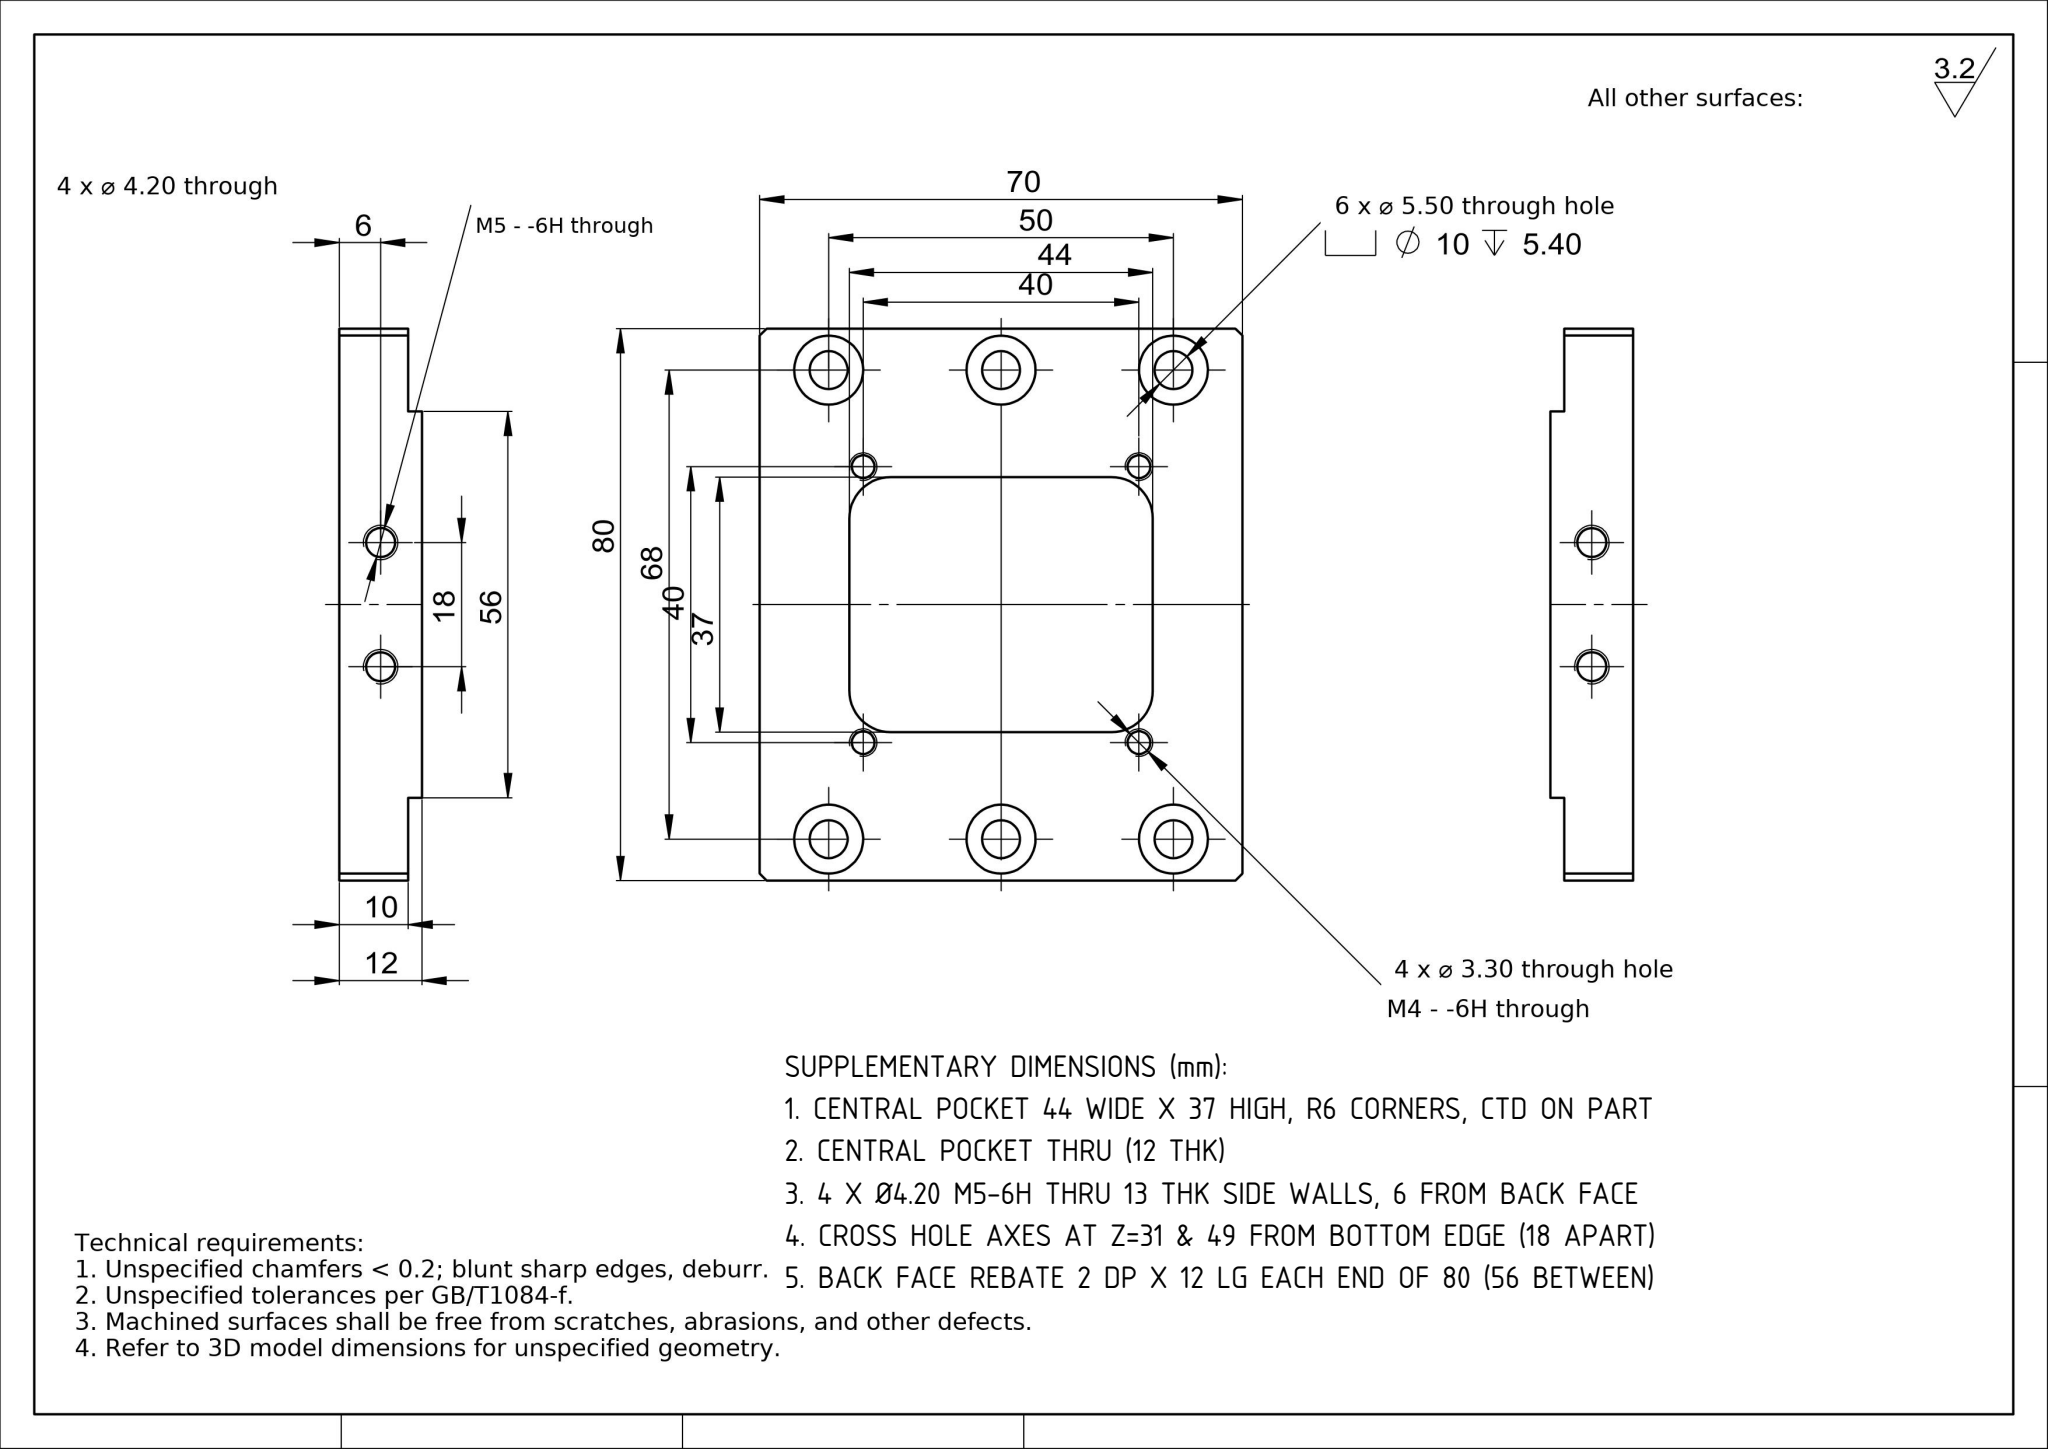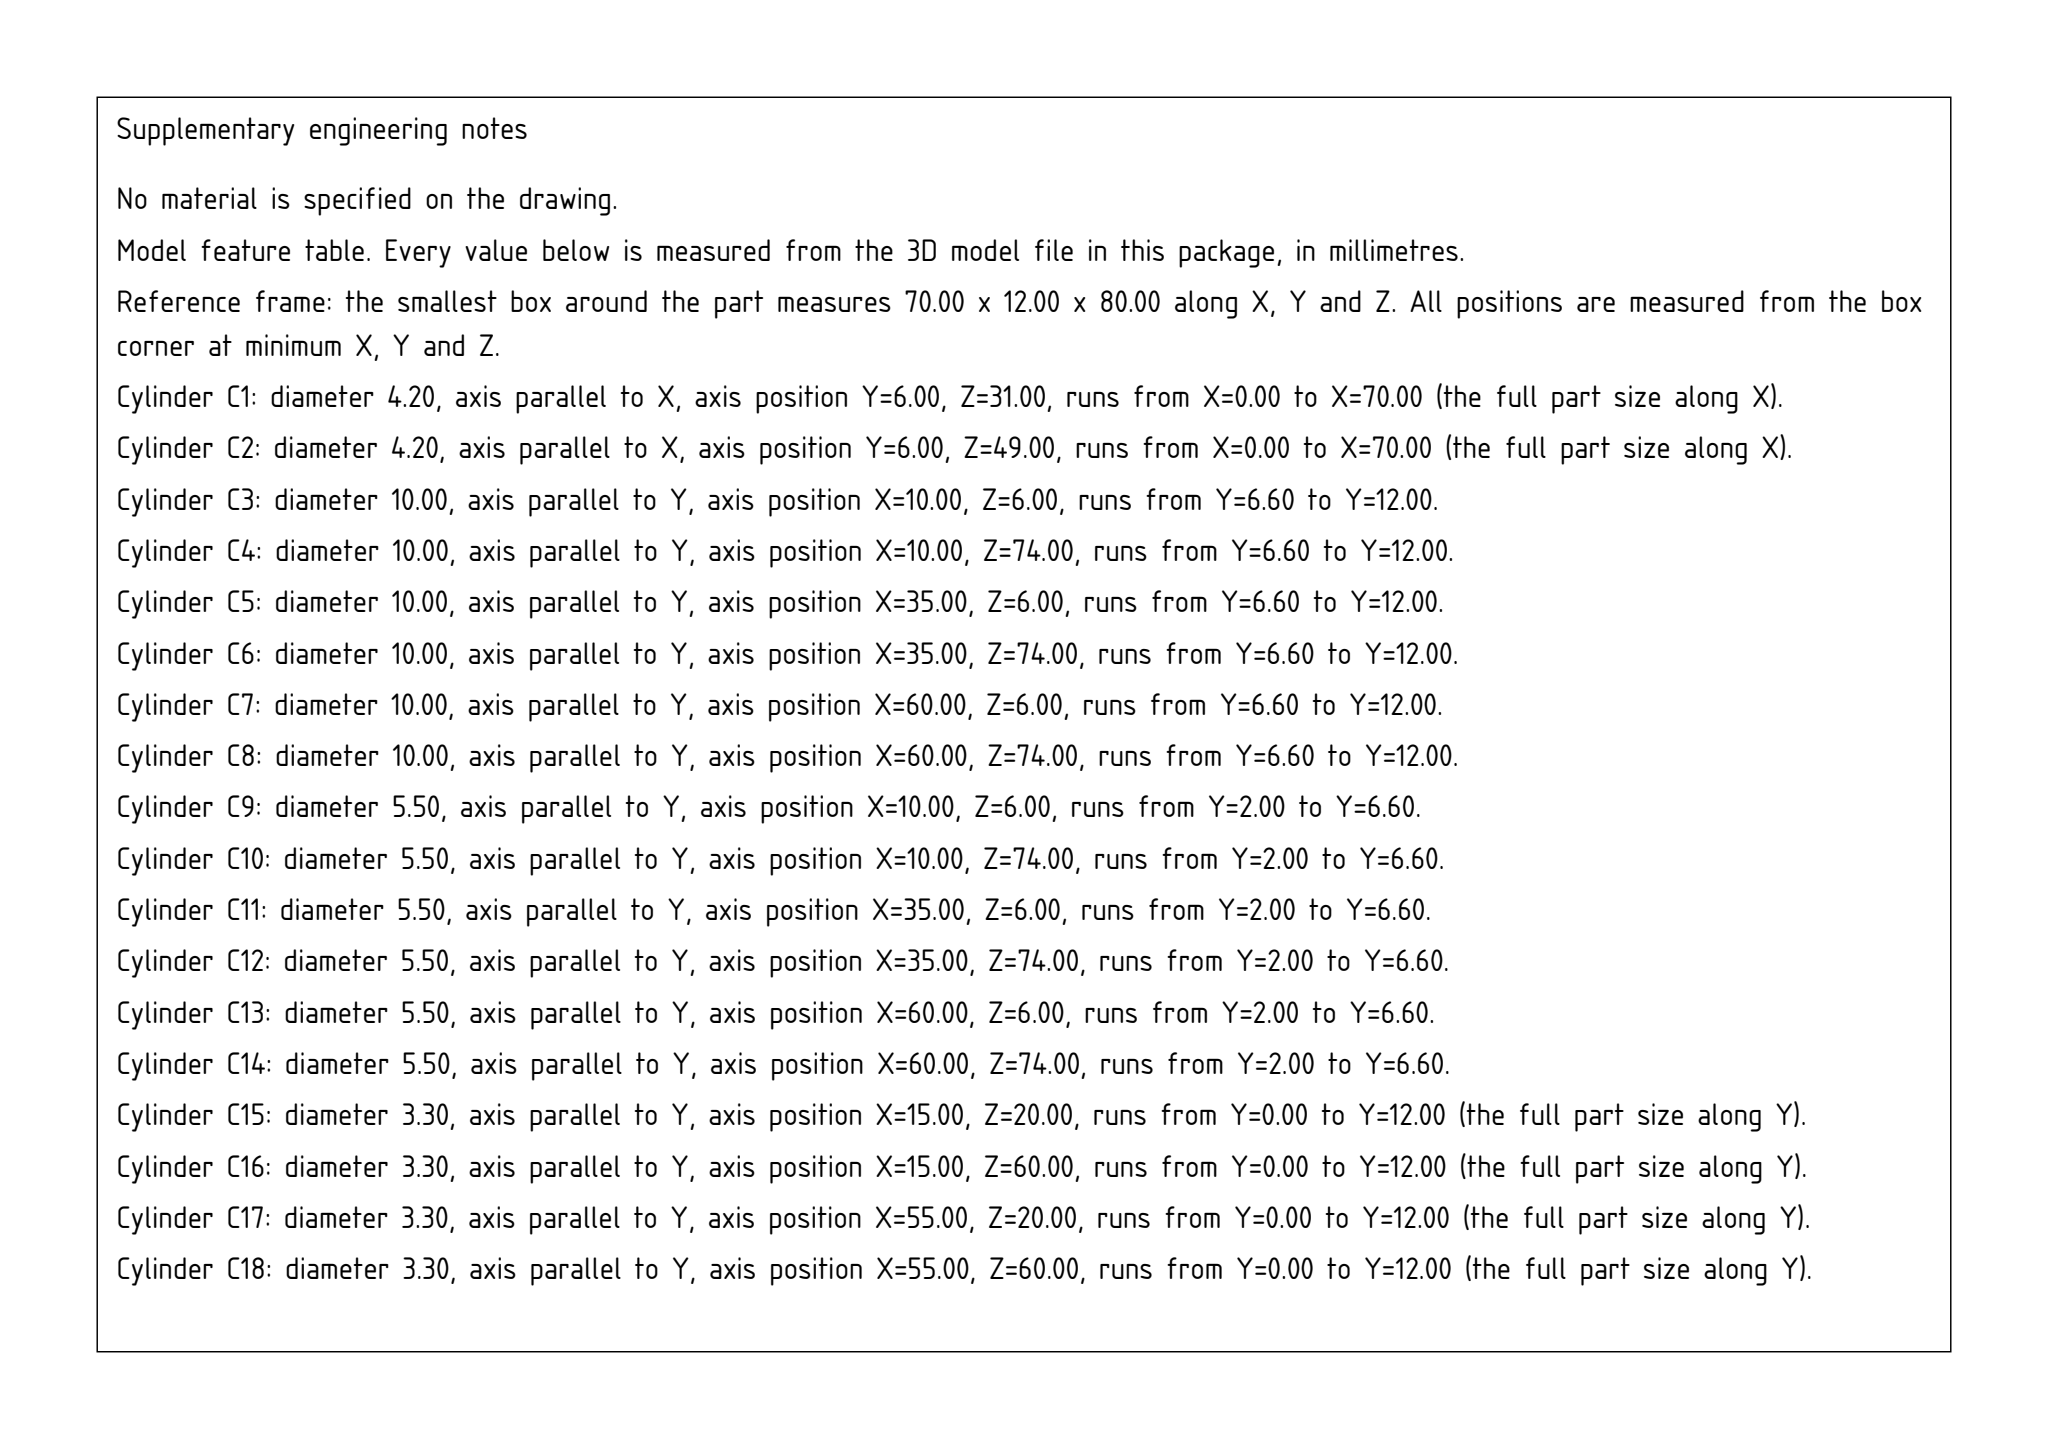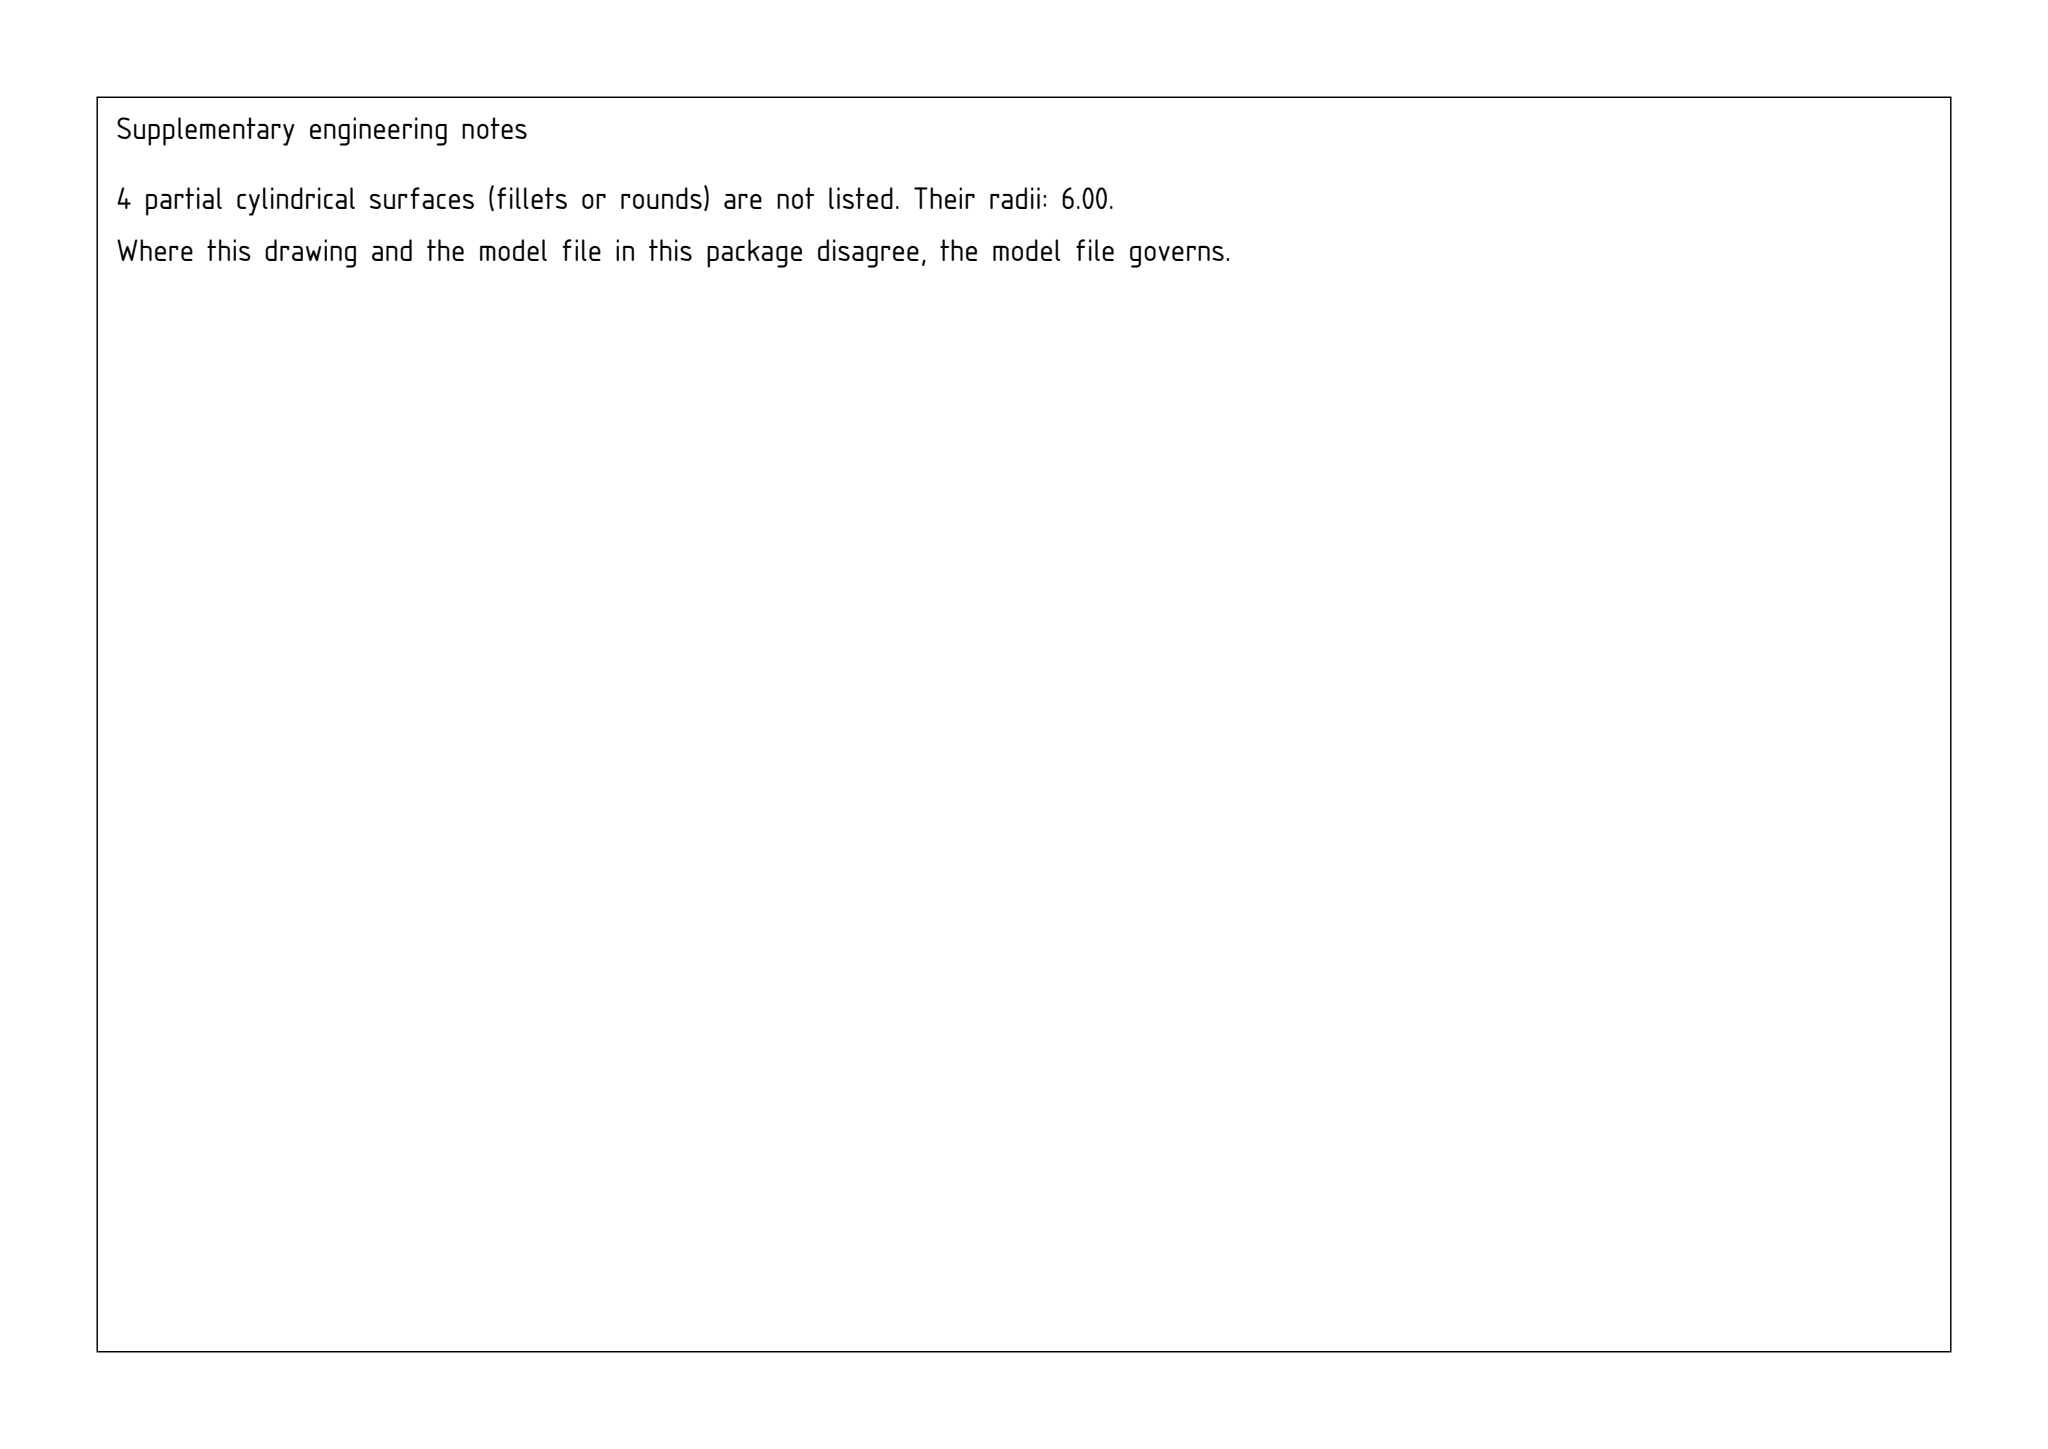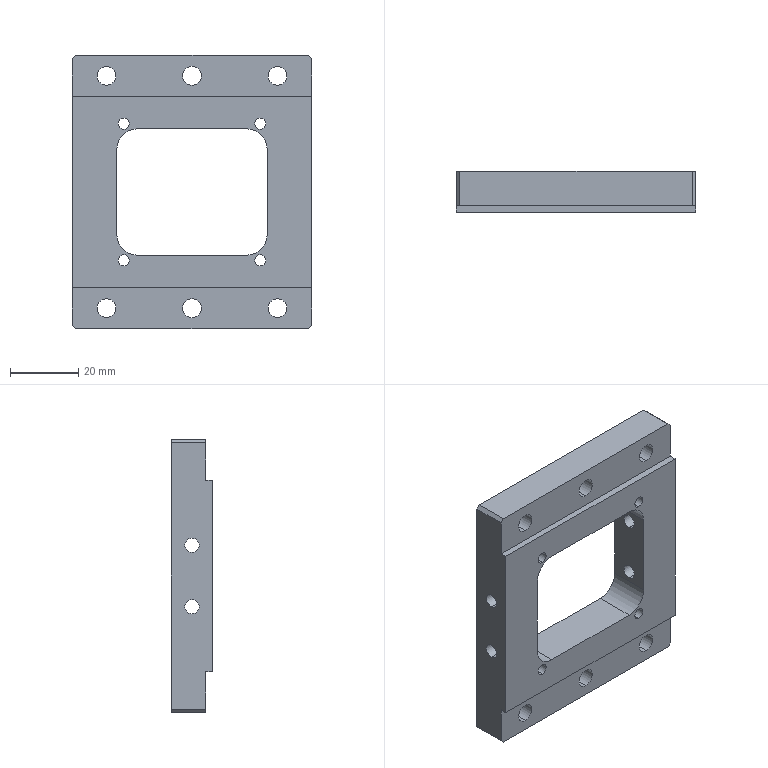Part | SolidWorks | mm | 1 solid | 68 faces | box 70 x 12 x 80 mm | volume 40323 mm3 | cylinder 44 | plane 24 | commonest cylinder face diameters 10 x12 5.5 x12 4.2 x8 3.3 x8 12 x4
build123d program:
from build123d import *

# Parameters (mm, degrees)
SKETCH1_W                                       = 70
SKETCH1_H                                       = 80
BOSS_EXTRUDE1_DEPTH                             = 6
SKETCH2_W                                       = 44
SKETCH2_H                                       = 37
CUT_EXTRUDE1_DEPTH                              = 55.489
FILLET1_R                                       = 6
SKETCH3_W                                       = 70
SKETCH3_H                                       = 12
CUT_EXTRUDE2_DEPTH                              = 2
M4_TAPPED_HOLE1_D                               = 3.3
M5_HEX_SOCKET_HEAD_CAP_SCREW_CBORE1_D           = 5.5
M5_HEX_SOCKET_HEAD_CAP_SCREW_CBORE1_CBORE_D     = 10
M5_HEX_SOCKET_HEAD_CAP_SCREW_CBORE1_CBORE_DEPTH = 5.4
CHAMFER1_SIZE                                   = 1
M5_TAPPED_HOLE1_REACH                           = 82.846
M5_TAPPED_HOLE1_BORE_R                          = 2.1


with BuildPart() as part:
    # Sketch1 → Boss-Extrude1 (new, symmetric)
    with BuildSketch(Plane(origin=(0, 0, 0), x_dir=(1, 0, 0), z_dir=(0, 1, 0))):
        Rectangle(SKETCH1_W, SKETCH1_H)
    extrude(amount=BOSS_EXTRUDE1_DEPTH, both=True)

    # Sketch2 → Cut-Extrude1 (cut, through all)
    with BuildSketch(Plane(origin=(0, 6, 0), x_dir=(1, 0, 0), z_dir=(0, 1, 0))):
        Rectangle(SKETCH2_W, SKETCH2_H)
    extrude(amount=-CUT_EXTRUDE1_DEPTH, mode=Mode.SUBTRACT)

    # Fillet1
    fillet1_edges = [part.edges().sort_by_distance(p)[0] for p in [
        (22, 0, -18.5),
        (22, 0, 18.5),
        (-22, 0, 18.5),
        (-22, 0, -18.5),
    ]]
    fillet(fillet1_edges, radius=FILLET1_R)

    # Sketch3 → Cut-Extrude2 (cut)
    with BuildSketch(Plane.XZ.offset(6)):
        with Locations((0, 34)):
            Rectangle(SKETCH3_W, SKETCH3_H)
        with Locations((0, -34)):
            Rectangle(SKETCH3_W, SKETCH3_H)
    extrude(amount=-CUT_EXTRUDE2_DEPTH, mode=Mode.SUBTRACT)

    # M4 Tapped Hole1 (through all)
    with Locations(Plane(origin=(0, 6, 0), x_dir=(1, 0, 0), z_dir=(0, 1, 0))):
        with Locations((-20, 20), (20, 20), (20, -20), (-20, -20)):
            Hole(M4_TAPPED_HOLE1_D / 2)

    # M5 Hex Socket Head Cap Screw CBORE1 (through all)
    with Locations(Plane(origin=(0, 6, 0), x_dir=(1, 0, 0), z_dir=(0, 1, 0))):
        with Locations((-25, 34), (0, 34), (25, 34), (25, -34), (0, -34), (-25, -34)):
            CounterBoreHole(M5_HEX_SOCKET_HEAD_CAP_SCREW_CBORE1_D / 2, M5_HEX_SOCKET_HEAD_CAP_SCREW_CBORE1_CBORE_D / 2, M5_HEX_SOCKET_HEAD_CAP_SCREW_CBORE1_CBORE_DEPTH)

    # Chamfer1
    chamfer1_edges = [part.edges().sort_by_distance(p)[0] for p in [
        (35, 1, 40),
        (-35, 1, 40),
        (-35, 1, -40),
        (35, 1, -40),
    ]]
    chamfer(chamfer1_edges, length=CHAMFER1_SIZE)

    # M5 Tapped Hole1 bore → M5 Tapped Hole1 (cut, up to next)
    with BuildSketch(Plane.ZY.offset(35), mode=Mode.PRIVATE) as m5_tapped_hole1_sk1:
        with Locations((-9, 0)):
            Circle(M5_TAPPED_HOLE1_BORE_R)
    m5_tapped_hole1_tool1 = extrude(m5_tapped_hole1_sk1.sketch, amount=-M5_TAPPED_HOLE1_REACH, mode=Mode.PRIVATE) & part.part
    # M5 Tapped Hole1 bore → M5 Tapped Hole1 (cut, up to next)
    with BuildSketch(Plane.ZY.offset(35), mode=Mode.PRIVATE) as m5_tapped_hole1_sk2:
        with Locations((9, 0)):
            Circle(M5_TAPPED_HOLE1_BORE_R)
    m5_tapped_hole1_tool2 = extrude(m5_tapped_hole1_sk2.sketch, amount=-M5_TAPPED_HOLE1_REACH, mode=Mode.PRIVATE) & part.part
    m5_tapped_hole1_1 = m5_tapped_hole1_tool1.solids().sort_by_distance((-35, 0, -9))[0]
    add(m5_tapped_hole1_1, mode=Mode.SUBTRACT)
    m5_tapped_hole1_2 = m5_tapped_hole1_tool2.solids().sort_by_distance((-35, 0, 9))[0]
    add(m5_tapped_hole1_2, mode=Mode.SUBTRACT)
    m5_tapped_hole1 = m5_tapped_hole1_1 + m5_tapped_hole1_2  # M5 Tapped Hole1 as one shape, for the pattern or mirror that repeats it

    # Mirror1: M5 Tapped Hole1 across plane
    add(m5_tapped_hole1.mirror(Plane(origin=(0, 0, 0), x_dir=(0, 0, 1), z_dir=(1, 0, 0))), mode=Mode.SUBTRACT)


solid = part.part